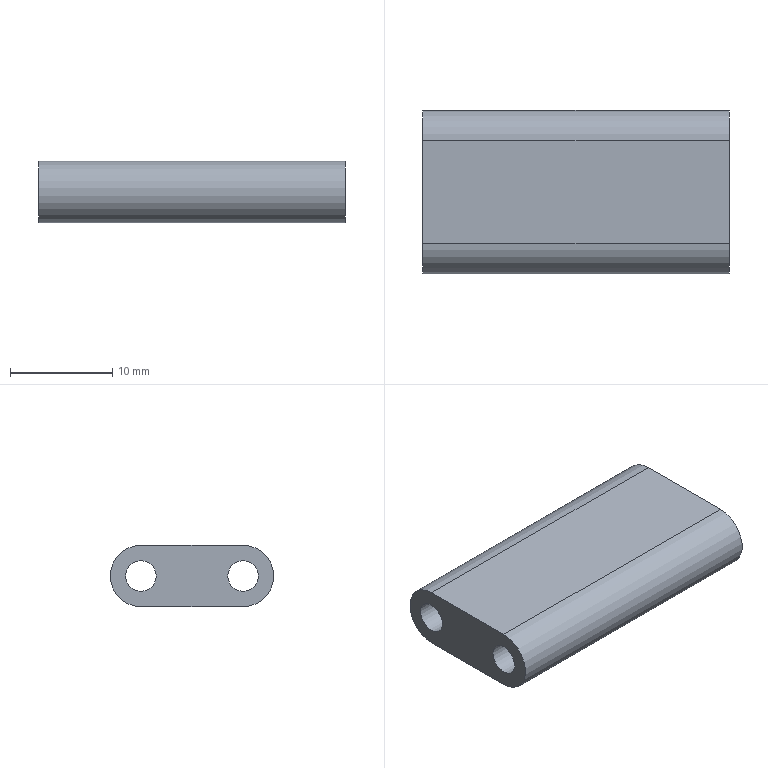Component | NX | PART_4_2 | 1 solid | 8 faces | box 30 x 16 x 6 mm | volume 2224 mm3 | cylinder 4 | plane 4 | commonest cylinder face diameters 6 x2 3 x2
STEP:
#1=CARTESIAN_POINT('',(0.,0.,0.));
#2=DIRECTION('',(0.,0.,1.));
#3=DIRECTION('',(1.,0.,0.));
#4=AXIS2_PLACEMENT_3D('',#1,#2,#3);
#5=CARTESIAN_POINT('',(-15.,1.,103.));
#6=VERTEX_POINT('',#5);
#7=CARTESIAN_POINT('',(-15.,1.,97.));
#8=VERTEX_POINT('',#7);
#9=CARTESIAN_POINT('',(-15.,1.,100.));
#10=DIRECTION('',(1.,0.,0.));
#11=DIRECTION('',(0.,1.,0.));
#12=AXIS2_PLACEMENT_3D('',#9,#10,#11);
#13=CIRCLE('',#12,3.);
#14=CARTESIAN_POINT('',(15.,1.,100.));
#15=DIRECTION('',(-1.,0.,0.));
#16=DIRECTION('',(0.,0.,1.));
#17=AXIS2_PLACEMENT_3D('',#14,#15,#16);
#18=CYLINDRICAL_SURFACE('',#17,3.);
#19=CARTESIAN_POINT('',(7.854,30.));
#20=DIRECTION('',(-1.,0.));
#21=VECTOR('',#20,1.);
#22=LINE('',#19,#21);
#23=(GEOMETRIC_REPRESENTATION_CONTEXT(2)PARAMETRIC_REPRESENTATION_CONTEXT()REPRESENTATION_CONTEXT('',''));
#24=DEFINITIONAL_REPRESENTATION('',(#22),#23);
#25=PCURVE('',#18,#24);
#26=CARTESIAN_POINT('',(-15.,1.,100.));
#27=DIRECTION('',(1.,0.,0.));
#28=DIRECTION('',(0.,0.,-1.));
#29=AXIS2_PLACEMENT_3D('',#26,#27,#28);
#30=PLANE('',#29);
#31=CARTESIAN_POINT('',(0.,0.));
#32=DIRECTION('',(0.,1.));
#33=AXIS2_PLACEMENT_2D('',#31,#32);
#34=CIRCLE('',#33,3.);
#35=(GEOMETRIC_REPRESENTATION_CONTEXT(2)PARAMETRIC_REPRESENTATION_CONTEXT()REPRESENTATION_CONTEXT('',''));
#36=DEFINITIONAL_REPRESENTATION('',(#34),#35);
#37=PCURVE('',#30,#36);
#38=SURFACE_CURVE('',#13,(#25,#37),.PCURVE_S1.);
#39=EDGE_CURVE('',#6,#8,#38,.T.);
#40=ORIENTED_EDGE('',*,*,#39,.T.);
#41=CARTESIAN_POINT('',(15.,1.,97.));
#42=VERTEX_POINT('',#41);
#43=CARTESIAN_POINT('',(15.,1.,97.));
#44=DIRECTION('',(-1.,0.,0.));
#45=VECTOR('',#44,1.);
#46=LINE('',#43,#45);
#47=CARTESIAN_POINT('',(3.142,0.));
#48=DIRECTION('',(0.,1.));
#49=VECTOR('',#48,1.);
#50=LINE('',#47,#49);
#51=(GEOMETRIC_REPRESENTATION_CONTEXT(2)PARAMETRIC_REPRESENTATION_CONTEXT()REPRESENTATION_CONTEXT('',''));
#52=DEFINITIONAL_REPRESENTATION('',(#50),#51);
#53=PCURVE('',#18,#52);
#54=CARTESIAN_POINT('',(15.,1.,97.));
#55=DIRECTION('',(0.,0.,1.));
#56=DIRECTION('',(1.,0.,0.));
#57=AXIS2_PLACEMENT_3D('',#54,#55,#56);
#58=PLANE('',#57);
#59=CARTESIAN_POINT('',(0.,0.));
#60=DIRECTION('',(-1.,0.));
#61=VECTOR('',#60,1.);
#62=LINE('',#59,#61);
#63=(GEOMETRIC_REPRESENTATION_CONTEXT(2)PARAMETRIC_REPRESENTATION_CONTEXT()REPRESENTATION_CONTEXT('',''));
#64=DEFINITIONAL_REPRESENTATION('',(#62),#63);
#65=PCURVE('',#58,#64);
#66=SURFACE_CURVE('',#46,(#53,#65),.PCURVE_S1.);
#67=EDGE_CURVE('',#42,#8,#66,.T.);
#68=ORIENTED_EDGE('',*,*,#67,.F.);
#69=CARTESIAN_POINT('',(15.,1.,103.));
#70=VERTEX_POINT('',#69);
#71=CARTESIAN_POINT('',(15.,1.,100.));
#72=DIRECTION('',(1.,0.,0.));
#73=DIRECTION('',(0.,1.,0.));
#74=AXIS2_PLACEMENT_3D('',#71,#72,#73);
#75=CIRCLE('',#74,3.);
#76=CARTESIAN_POINT('',(7.854,0.));
#77=DIRECTION('',(-1.,0.));
#78=VECTOR('',#77,1.);
#79=LINE('',#76,#78);
#80=(GEOMETRIC_REPRESENTATION_CONTEXT(2)PARAMETRIC_REPRESENTATION_CONTEXT()REPRESENTATION_CONTEXT('',''));
#81=DEFINITIONAL_REPRESENTATION('',(#79),#80);
#82=PCURVE('',#18,#81);
#83=CARTESIAN_POINT('',(15.,1.,100.));
#84=DIRECTION('',(1.,0.,0.));
#85=DIRECTION('',(0.,0.,-1.));
#86=AXIS2_PLACEMENT_3D('',#83,#84,#85);
#87=PLANE('',#86);
#88=CARTESIAN_POINT('',(0.,0.));
#89=DIRECTION('',(0.,1.));
#90=AXIS2_PLACEMENT_2D('',#88,#89);
#91=CIRCLE('',#90,3.);
#92=(GEOMETRIC_REPRESENTATION_CONTEXT(2)PARAMETRIC_REPRESENTATION_CONTEXT()REPRESENTATION_CONTEXT('',''));
#93=DEFINITIONAL_REPRESENTATION('',(#91),#92);
#94=PCURVE('',#87,#93);
#95=SURFACE_CURVE('',#75,(#82,#94),.PCURVE_S1.);
#96=EDGE_CURVE('',#70,#42,#95,.T.);
#97=ORIENTED_EDGE('',*,*,#96,.F.);
#98=CARTESIAN_POINT('',(15.,1.,103.));
#99=DIRECTION('',(-1.,0.,0.));
#100=VECTOR('',#99,1.);
#101=LINE('',#98,#100);
#102=CARTESIAN_POINT('',(6.283,0.));
#103=DIRECTION('',(0.,1.));
#104=VECTOR('',#103,1.);
#105=LINE('',#102,#104);
#106=(GEOMETRIC_REPRESENTATION_CONTEXT(2)PARAMETRIC_REPRESENTATION_CONTEXT()REPRESENTATION_CONTEXT('',''));
#107=DEFINITIONAL_REPRESENTATION('',(#105),#106);
#108=PCURVE('',#18,#107);
#109=CARTESIAN_POINT('',(15.,11.,103.));
#110=DIRECTION('',(0.,0.,-1.));
#111=DIRECTION('',(-1.,0.,0.));
#112=AXIS2_PLACEMENT_3D('',#109,#110,#111);
#113=PLANE('',#112);
#114=CARTESIAN_POINT('',(0.,-10.));
#115=DIRECTION('',(1.,0.));
#116=VECTOR('',#115,1.);
#117=LINE('',#114,#116);
#118=(GEOMETRIC_REPRESENTATION_CONTEXT(2)PARAMETRIC_REPRESENTATION_CONTEXT()REPRESENTATION_CONTEXT('',''));
#119=DEFINITIONAL_REPRESENTATION('',(#117),#118);
#120=PCURVE('',#113,#119);
#121=SURFACE_CURVE('',#101,(#108,#120),.PCURVE_S1.);
#122=EDGE_CURVE('',#70,#6,#121,.T.);
#123=ORIENTED_EDGE('',*,*,#122,.T.);
#124=EDGE_LOOP('',(#40,#68,#97,#123));
#125=FACE_BOUND('',#124,.T.);
#126=ADVANCED_FACE('',(#125),#18,.T.);
#127=CARTESIAN_POINT('',(-15.,11.,97.));
#128=VERTEX_POINT('',#127);
#129=CARTESIAN_POINT('',(-15.,1.,97.));
#130=DIRECTION('',(0.,1.,0.));
#131=VECTOR('',#130,1.);
#132=LINE('',#129,#131);
#133=CARTESIAN_POINT('',(-30.,0.));
#134=DIRECTION('',(0.,1.));
#135=VECTOR('',#134,1.);
#136=LINE('',#133,#135);
#137=(GEOMETRIC_REPRESENTATION_CONTEXT(2)PARAMETRIC_REPRESENTATION_CONTEXT()REPRESENTATION_CONTEXT('',''));
#138=DEFINITIONAL_REPRESENTATION('',(#136),#137);
#139=PCURVE('',#58,#138);
#140=CARTESIAN_POINT('',(3.,0.));
#141=DIRECTION('',(0.,1.));
#142=VECTOR('',#141,1.);
#143=LINE('',#140,#142);
#144=(GEOMETRIC_REPRESENTATION_CONTEXT(2)PARAMETRIC_REPRESENTATION_CONTEXT()REPRESENTATION_CONTEXT('',''));
#145=DEFINITIONAL_REPRESENTATION('',(#143),#144);
#146=PCURVE('',#30,#145);
#147=SURFACE_CURVE('',#132,(#139,#146),.PCURVE_S1.);
#148=EDGE_CURVE('',#8,#128,#147,.T.);
#149=ORIENTED_EDGE('',*,*,#148,.T.);
#150=CARTESIAN_POINT('',(15.,11.,97.));
#151=VERTEX_POINT('',#150);
#152=CARTESIAN_POINT('',(15.,11.,97.));
#153=DIRECTION('',(-1.,0.,0.));
#154=VECTOR('',#153,1.);
#155=LINE('',#152,#154);
#156=CARTESIAN_POINT('',(0.,10.));
#157=DIRECTION('',(-1.,0.));
#158=VECTOR('',#157,1.);
#159=LINE('',#156,#158);
#160=(GEOMETRIC_REPRESENTATION_CONTEXT(2)PARAMETRIC_REPRESENTATION_CONTEXT()REPRESENTATION_CONTEXT('',''));
#161=DEFINITIONAL_REPRESENTATION('',(#159),#160);
#162=PCURVE('',#58,#161);
#163=CARTESIAN_POINT('',(15.,11.,100.));
#164=DIRECTION('',(-1.,0.,0.));
#165=DIRECTION('',(0.,0.,1.));
#166=AXIS2_PLACEMENT_3D('',#163,#164,#165);
#167=CYLINDRICAL_SURFACE('',#166,3.);
#168=CARTESIAN_POINT('',(3.142,0.));
#169=DIRECTION('',(0.,1.));
#170=VECTOR('',#169,1.);
#171=LINE('',#168,#170);
#172=(GEOMETRIC_REPRESENTATION_CONTEXT(2)PARAMETRIC_REPRESENTATION_CONTEXT()REPRESENTATION_CONTEXT('',''));
#173=DEFINITIONAL_REPRESENTATION('',(#171),#172);
#174=PCURVE('',#167,#173);
#175=SURFACE_CURVE('',#155,(#162,#174),.PCURVE_S1.);
#176=EDGE_CURVE('',#151,#128,#175,.T.);
#177=ORIENTED_EDGE('',*,*,#176,.F.);
#178=CARTESIAN_POINT('',(15.,1.,97.));
#179=DIRECTION('',(0.,1.,0.));
#180=VECTOR('',#179,1.);
#181=LINE('',#178,#180);
#182=CARTESIAN_POINT('',(0.,0.));
#183=DIRECTION('',(0.,1.));
#184=VECTOR('',#183,1.);
#185=LINE('',#182,#184);
#186=(GEOMETRIC_REPRESENTATION_CONTEXT(2)PARAMETRIC_REPRESENTATION_CONTEXT()REPRESENTATION_CONTEXT('',''));
#187=DEFINITIONAL_REPRESENTATION('',(#185),#186);
#188=PCURVE('',#58,#187);
#189=CARTESIAN_POINT('',(3.,0.));
#190=DIRECTION('',(0.,1.));
#191=VECTOR('',#190,1.);
#192=LINE('',#189,#191);
#193=(GEOMETRIC_REPRESENTATION_CONTEXT(2)PARAMETRIC_REPRESENTATION_CONTEXT()REPRESENTATION_CONTEXT('',''));
#194=DEFINITIONAL_REPRESENTATION('',(#192),#193);
#195=PCURVE('',#87,#194);
#196=SURFACE_CURVE('',#181,(#188,#195),.PCURVE_S1.);
#197=EDGE_CURVE('',#42,#151,#196,.T.);
#198=ORIENTED_EDGE('',*,*,#197,.F.);
#199=ORIENTED_EDGE('',*,*,#67,.T.);
#200=EDGE_LOOP('',(#149,#177,#198,#199));
#201=FACE_BOUND('',#200,.T.);
#202=ADVANCED_FACE('',(#201),#58,.F.);
#203=CARTESIAN_POINT('',(-15.,11.,103.));
#204=VERTEX_POINT('',#203);
#205=CARTESIAN_POINT('',(-15.,11.,100.));
#206=DIRECTION('',(1.,0.,0.));
#207=DIRECTION('',(0.,1.,0.));
#208=AXIS2_PLACEMENT_3D('',#205,#206,#207);
#209=CIRCLE('',#208,3.);
#210=CARTESIAN_POINT('',(7.854,30.));
#211=DIRECTION('',(-1.,0.));
#212=VECTOR('',#211,1.);
#213=LINE('',#210,#212);
#214=(GEOMETRIC_REPRESENTATION_CONTEXT(2)PARAMETRIC_REPRESENTATION_CONTEXT()REPRESENTATION_CONTEXT('',''));
#215=DEFINITIONAL_REPRESENTATION('',(#213),#214);
#216=PCURVE('',#167,#215);
#217=CARTESIAN_POINT('',(0.,10.));
#218=DIRECTION('',(0.,1.));
#219=AXIS2_PLACEMENT_2D('',#217,#218);
#220=CIRCLE('',#219,3.);
#221=(GEOMETRIC_REPRESENTATION_CONTEXT(2)PARAMETRIC_REPRESENTATION_CONTEXT()REPRESENTATION_CONTEXT('',''));
#222=DEFINITIONAL_REPRESENTATION('',(#220),#221);
#223=PCURVE('',#30,#222);
#224=SURFACE_CURVE('',#209,(#216,#223),.PCURVE_S1.);
#225=EDGE_CURVE('',#128,#204,#224,.T.);
#226=ORIENTED_EDGE('',*,*,#225,.T.);
#227=CARTESIAN_POINT('',(15.,11.,103.));
#228=VERTEX_POINT('',#227);
#229=CARTESIAN_POINT('',(15.,11.,103.));
#230=DIRECTION('',(-1.,0.,0.));
#231=VECTOR('',#230,1.);
#232=LINE('',#229,#231);
#233=CARTESIAN_POINT('',(0.,0.));
#234=DIRECTION('',(0.,1.));
#235=VECTOR('',#234,1.);
#236=LINE('',#233,#235);
#237=(GEOMETRIC_REPRESENTATION_CONTEXT(2)PARAMETRIC_REPRESENTATION_CONTEXT()REPRESENTATION_CONTEXT('',''));
#238=DEFINITIONAL_REPRESENTATION('',(#236),#237);
#239=PCURVE('',#167,#238);
#240=CARTESIAN_POINT('',(0.,0.));
#241=DIRECTION('',(1.,0.));
#242=VECTOR('',#241,1.);
#243=LINE('',#240,#242);
#244=(GEOMETRIC_REPRESENTATION_CONTEXT(2)PARAMETRIC_REPRESENTATION_CONTEXT()REPRESENTATION_CONTEXT('',''));
#245=DEFINITIONAL_REPRESENTATION('',(#243),#244);
#246=PCURVE('',#113,#245);
#247=SURFACE_CURVE('',#232,(#239,#246),.PCURVE_S1.);
#248=EDGE_CURVE('',#228,#204,#247,.T.);
#249=ORIENTED_EDGE('',*,*,#248,.F.);
#250=CARTESIAN_POINT('',(15.,11.,100.));
#251=DIRECTION('',(1.,0.,0.));
#252=DIRECTION('',(0.,1.,0.));
#253=AXIS2_PLACEMENT_3D('',#250,#251,#252);
#254=CIRCLE('',#253,3.);
#255=CARTESIAN_POINT('',(7.854,0.));
#256=DIRECTION('',(-1.,0.));
#257=VECTOR('',#256,1.);
#258=LINE('',#255,#257);
#259=(GEOMETRIC_REPRESENTATION_CONTEXT(2)PARAMETRIC_REPRESENTATION_CONTEXT()REPRESENTATION_CONTEXT('',''));
#260=DEFINITIONAL_REPRESENTATION('',(#258),#259);
#261=PCURVE('',#167,#260);
#262=CARTESIAN_POINT('',(0.,10.));
#263=DIRECTION('',(0.,1.));
#264=AXIS2_PLACEMENT_2D('',#262,#263);
#265=CIRCLE('',#264,3.);
#266=(GEOMETRIC_REPRESENTATION_CONTEXT(2)PARAMETRIC_REPRESENTATION_CONTEXT()REPRESENTATION_CONTEXT('',''));
#267=DEFINITIONAL_REPRESENTATION('',(#265),#266);
#268=PCURVE('',#87,#267);
#269=SURFACE_CURVE('',#254,(#261,#268),.PCURVE_S1.);
#270=EDGE_CURVE('',#151,#228,#269,.T.);
#271=ORIENTED_EDGE('',*,*,#270,.F.);
#272=ORIENTED_EDGE('',*,*,#176,.T.);
#273=EDGE_LOOP('',(#226,#249,#271,#272));
#274=FACE_BOUND('',#273,.T.);
#275=ADVANCED_FACE('',(#274),#167,.T.);
#276=CARTESIAN_POINT('',(15.,2.5,100.));
#277=VERTEX_POINT('',#276);
#278=CARTESIAN_POINT('',(15.,1.,100.));
#279=DIRECTION('',(1.,0.,0.));
#280=DIRECTION('',(0.,1.,0.));
#281=AXIS2_PLACEMENT_3D('',#278,#279,#280);
#282=CIRCLE('',#281,1.5);
#283=CARTESIAN_POINT('',(15.,1.,100.));
#284=DIRECTION('',(-1.,0.,0.));
#285=DIRECTION('',(0.,0.,1.));
#286=AXIS2_PLACEMENT_3D('',#283,#284,#285);
#287=CYLINDRICAL_SURFACE('',#286,1.5);
#288=CARTESIAN_POINT('',(7.854,0.));
#289=DIRECTION('',(-1.,0.));
#290=VECTOR('',#289,1.);
#291=LINE('',#288,#290);
#292=(GEOMETRIC_REPRESENTATION_CONTEXT(2)PARAMETRIC_REPRESENTATION_CONTEXT()REPRESENTATION_CONTEXT('',''));
#293=DEFINITIONAL_REPRESENTATION('',(#291),#292);
#294=PCURVE('',#287,#293);
#295=CARTESIAN_POINT('',(0.,0.));
#296=DIRECTION('',(0.,1.));
#297=AXIS2_PLACEMENT_2D('',#295,#296);
#298=CIRCLE('',#297,1.5);
#299=(GEOMETRIC_REPRESENTATION_CONTEXT(2)PARAMETRIC_REPRESENTATION_CONTEXT()REPRESENTATION_CONTEXT('',''));
#300=DEFINITIONAL_REPRESENTATION('',(#298),#299);
#301=PCURVE('',#87,#300);
#302=SURFACE_CURVE('',#282,(#294,#301),.PCURVE_S1.);
#303=EDGE_CURVE('',#277,#277,#302,.T.);
#304=ORIENTED_EDGE('',*,*,#303,.F.);
#305=CARTESIAN_POINT('',(-15.,2.5,100.));
#306=VERTEX_POINT('',#305);
#307=CARTESIAN_POINT('',(15.,2.5,100.));
#308=CARTESIAN_POINT('',(-15.,2.5,100.));
#309=B_SPLINE_CURVE_WITH_KNOTS('',1,(#307,#308),.UNSPECIFIED.,.F.,.F.,(2,2),(0.,30.),.PIECEWISE_BEZIER_KNOTS.);
#310=CARTESIAN_POINT('',(7.854,0.));
#311=DIRECTION('',(0.,1.));
#312=VECTOR('',#311,1.);
#313=LINE('',#310,#312);
#314=(GEOMETRIC_REPRESENTATION_CONTEXT(2)PARAMETRIC_REPRESENTATION_CONTEXT()REPRESENTATION_CONTEXT('',''));
#315=DEFINITIONAL_REPRESENTATION('',(#313),#314);
#316=PCURVE('',#287,#315);
#317=CARTESIAN_POINT('',(1.571,0.));
#318=DIRECTION('',(0.,1.));
#319=VECTOR('',#318,1.);
#320=LINE('',#317,#319);
#321=(GEOMETRIC_REPRESENTATION_CONTEXT(2)PARAMETRIC_REPRESENTATION_CONTEXT()REPRESENTATION_CONTEXT('',''));
#322=DEFINITIONAL_REPRESENTATION('',(#320),#321);
#323=PCURVE('',#287,#322);
#324=SEAM_CURVE('',#309,(#316,#323),.PCURVE_S1.);
#325=EDGE_CURVE('',#277,#306,#324,.T.);
#326=ORIENTED_EDGE('',*,*,#325,.T.);
#327=CARTESIAN_POINT('',(-15.,1.,100.));
#328=DIRECTION('',(1.,0.,0.));
#329=DIRECTION('',(0.,1.,0.));
#330=AXIS2_PLACEMENT_3D('',#327,#328,#329);
#331=CIRCLE('',#330,1.5);
#332=CARTESIAN_POINT('',(7.854,30.));
#333=DIRECTION('',(-1.,0.));
#334=VECTOR('',#333,1.);
#335=LINE('',#332,#334);
#336=(GEOMETRIC_REPRESENTATION_CONTEXT(2)PARAMETRIC_REPRESENTATION_CONTEXT()REPRESENTATION_CONTEXT('',''));
#337=DEFINITIONAL_REPRESENTATION('',(#335),#336);
#338=PCURVE('',#287,#337);
#339=CARTESIAN_POINT('',(0.,0.));
#340=DIRECTION('',(0.,1.));
#341=AXIS2_PLACEMENT_2D('',#339,#340);
#342=CIRCLE('',#341,1.5);
#343=(GEOMETRIC_REPRESENTATION_CONTEXT(2)PARAMETRIC_REPRESENTATION_CONTEXT()REPRESENTATION_CONTEXT('',''));
#344=DEFINITIONAL_REPRESENTATION('',(#342),#343);
#345=PCURVE('',#30,#344);
#346=SURFACE_CURVE('',#331,(#338,#345),.PCURVE_S1.);
#347=EDGE_CURVE('',#306,#306,#346,.T.);
#348=ORIENTED_EDGE('',*,*,#347,.T.);
#349=ORIENTED_EDGE('',*,*,#325,.F.);
#350=EDGE_LOOP('',(#304,#326,#348,#349));
#351=FACE_BOUND('',#350,.F.);
#352=ADVANCED_FACE('',(#351),#287,.F.);
#353=CARTESIAN_POINT('',(-15.,11.,103.));
#354=DIRECTION('',(0.,-1.,0.));
#355=VECTOR('',#354,1.);
#356=LINE('',#353,#355);
#357=CARTESIAN_POINT('',(30.,0.));
#358=DIRECTION('',(0.,-1.));
#359=VECTOR('',#358,1.);
#360=LINE('',#357,#359);
#361=(GEOMETRIC_REPRESENTATION_CONTEXT(2)PARAMETRIC_REPRESENTATION_CONTEXT()REPRESENTATION_CONTEXT('',''));
#362=DEFINITIONAL_REPRESENTATION('',(#360),#361);
#363=PCURVE('',#113,#362);
#364=CARTESIAN_POINT('',(-3.,10.));
#365=DIRECTION('',(0.,-1.));
#366=VECTOR('',#365,1.);
#367=LINE('',#364,#366);
#368=(GEOMETRIC_REPRESENTATION_CONTEXT(2)PARAMETRIC_REPRESENTATION_CONTEXT()REPRESENTATION_CONTEXT('',''));
#369=DEFINITIONAL_REPRESENTATION('',(#367),#368);
#370=PCURVE('',#30,#369);
#371=SURFACE_CURVE('',#356,(#363,#370),.PCURVE_S1.);
#372=EDGE_CURVE('',#204,#6,#371,.T.);
#373=ORIENTED_EDGE('',*,*,#372,.T.);
#374=ORIENTED_EDGE('',*,*,#122,.F.);
#375=CARTESIAN_POINT('',(15.,11.,103.));
#376=DIRECTION('',(0.,-1.,0.));
#377=VECTOR('',#376,1.);
#378=LINE('',#375,#377);
#379=CARTESIAN_POINT('',(0.,0.));
#380=DIRECTION('',(0.,-1.));
#381=VECTOR('',#380,1.);
#382=LINE('',#379,#381);
#383=(GEOMETRIC_REPRESENTATION_CONTEXT(2)PARAMETRIC_REPRESENTATION_CONTEXT()REPRESENTATION_CONTEXT('',''));
#384=DEFINITIONAL_REPRESENTATION('',(#382),#383);
#385=PCURVE('',#113,#384);
#386=CARTESIAN_POINT('',(-3.,10.));
#387=DIRECTION('',(0.,-1.));
#388=VECTOR('',#387,1.);
#389=LINE('',#386,#388);
#390=(GEOMETRIC_REPRESENTATION_CONTEXT(2)PARAMETRIC_REPRESENTATION_CONTEXT()REPRESENTATION_CONTEXT('',''));
#391=DEFINITIONAL_REPRESENTATION('',(#389),#390);
#392=PCURVE('',#87,#391);
#393=SURFACE_CURVE('',#378,(#385,#392),.PCURVE_S1.);
#394=EDGE_CURVE('',#228,#70,#393,.T.);
#395=ORIENTED_EDGE('',*,*,#394,.F.);
#396=ORIENTED_EDGE('',*,*,#248,.T.);
#397=EDGE_LOOP('',(#373,#374,#395,#396));
#398=FACE_BOUND('',#397,.T.);
#399=ADVANCED_FACE('',(#398),#113,.F.);
#400=CARTESIAN_POINT('',(15.,12.5,100.));
#401=VERTEX_POINT('',#400);
#402=CARTESIAN_POINT('',(15.,11.,100.));
#403=DIRECTION('',(1.,0.,0.));
#404=DIRECTION('',(0.,1.,0.));
#405=AXIS2_PLACEMENT_3D('',#402,#403,#404);
#406=CIRCLE('',#405,1.5);
#407=CARTESIAN_POINT('',(15.,11.,100.));
#408=DIRECTION('',(-1.,0.,0.));
#409=DIRECTION('',(0.,0.,1.));
#410=AXIS2_PLACEMENT_3D('',#407,#408,#409);
#411=CYLINDRICAL_SURFACE('',#410,1.5);
#412=CARTESIAN_POINT('',(7.854,0.));
#413=DIRECTION('',(-1.,0.));
#414=VECTOR('',#413,1.);
#415=LINE('',#412,#414);
#416=(GEOMETRIC_REPRESENTATION_CONTEXT(2)PARAMETRIC_REPRESENTATION_CONTEXT()REPRESENTATION_CONTEXT('',''));
#417=DEFINITIONAL_REPRESENTATION('',(#415),#416);
#418=PCURVE('',#411,#417);
#419=CARTESIAN_POINT('',(0.,10.));
#420=DIRECTION('',(0.,1.));
#421=AXIS2_PLACEMENT_2D('',#419,#420);
#422=CIRCLE('',#421,1.5);
#423=(GEOMETRIC_REPRESENTATION_CONTEXT(2)PARAMETRIC_REPRESENTATION_CONTEXT()REPRESENTATION_CONTEXT('',''));
#424=DEFINITIONAL_REPRESENTATION('',(#422),#423);
#425=PCURVE('',#87,#424);
#426=SURFACE_CURVE('',#406,(#418,#425),.PCURVE_S1.);
#427=EDGE_CURVE('',#401,#401,#426,.T.);
#428=ORIENTED_EDGE('',*,*,#427,.F.);
#429=CARTESIAN_POINT('',(-15.,12.5,100.));
#430=VERTEX_POINT('',#429);
#431=CARTESIAN_POINT('',(15.,12.5,100.));
#432=CARTESIAN_POINT('',(-15.,12.5,100.));
#433=B_SPLINE_CURVE_WITH_KNOTS('',1,(#431,#432),.UNSPECIFIED.,.F.,.F.,(2,2),(0.,30.),.PIECEWISE_BEZIER_KNOTS.);
#434=CARTESIAN_POINT('',(7.854,0.));
#435=DIRECTION('',(0.,1.));
#436=VECTOR('',#435,1.);
#437=LINE('',#434,#436);
#438=(GEOMETRIC_REPRESENTATION_CONTEXT(2)PARAMETRIC_REPRESENTATION_CONTEXT()REPRESENTATION_CONTEXT('',''));
#439=DEFINITIONAL_REPRESENTATION('',(#437),#438);
#440=PCURVE('',#411,#439);
#441=CARTESIAN_POINT('',(1.571,0.));
#442=DIRECTION('',(0.,1.));
#443=VECTOR('',#442,1.);
#444=LINE('',#441,#443);
#445=(GEOMETRIC_REPRESENTATION_CONTEXT(2)PARAMETRIC_REPRESENTATION_CONTEXT()REPRESENTATION_CONTEXT('',''));
#446=DEFINITIONAL_REPRESENTATION('',(#444),#445);
#447=PCURVE('',#411,#446);
#448=SEAM_CURVE('',#433,(#440,#447),.PCURVE_S1.);
#449=EDGE_CURVE('',#401,#430,#448,.T.);
#450=ORIENTED_EDGE('',*,*,#449,.T.);
#451=CARTESIAN_POINT('',(-15.,11.,100.));
#452=DIRECTION('',(1.,0.,0.));
#453=DIRECTION('',(0.,1.,0.));
#454=AXIS2_PLACEMENT_3D('',#451,#452,#453);
#455=CIRCLE('',#454,1.5);
#456=CARTESIAN_POINT('',(7.854,30.));
#457=DIRECTION('',(-1.,0.));
#458=VECTOR('',#457,1.);
#459=LINE('',#456,#458);
#460=(GEOMETRIC_REPRESENTATION_CONTEXT(2)PARAMETRIC_REPRESENTATION_CONTEXT()REPRESENTATION_CONTEXT('',''));
#461=DEFINITIONAL_REPRESENTATION('',(#459),#460);
#462=PCURVE('',#411,#461);
#463=CARTESIAN_POINT('',(0.,10.));
#464=DIRECTION('',(0.,1.));
#465=AXIS2_PLACEMENT_2D('',#463,#464);
#466=CIRCLE('',#465,1.5);
#467=(GEOMETRIC_REPRESENTATION_CONTEXT(2)PARAMETRIC_REPRESENTATION_CONTEXT()REPRESENTATION_CONTEXT('',''));
#468=DEFINITIONAL_REPRESENTATION('',(#466),#467);
#469=PCURVE('',#30,#468);
#470=SURFACE_CURVE('',#455,(#462,#469),.PCURVE_S1.);
#471=EDGE_CURVE('',#430,#430,#470,.T.);
#472=ORIENTED_EDGE('',*,*,#471,.T.);
#473=ORIENTED_EDGE('',*,*,#449,.F.);
#474=EDGE_LOOP('',(#428,#450,#472,#473));
#475=FACE_BOUND('',#474,.F.);
#476=ADVANCED_FACE('',(#475),#411,.F.);
#477=ORIENTED_EDGE('',*,*,#96,.T.);
#478=ORIENTED_EDGE('',*,*,#197,.T.);
#479=ORIENTED_EDGE('',*,*,#270,.T.);
#480=ORIENTED_EDGE('',*,*,#394,.T.);
#481=EDGE_LOOP('',(#477,#478,#479,#480));
#482=FACE_BOUND('',#481,.T.);
#483=ORIENTED_EDGE('',*,*,#303,.F.);
#484=EDGE_LOOP('',(#483));
#485=FACE_BOUND('',#484,.T.);
#486=ORIENTED_EDGE('',*,*,#427,.F.);
#487=EDGE_LOOP('',(#486));
#488=FACE_BOUND('',#487,.T.);
#489=ADVANCED_FACE('',(#482,#485,#488),#87,.T.);
#490=ORIENTED_EDGE('',*,*,#39,.F.);
#491=ORIENTED_EDGE('',*,*,#372,.F.);
#492=ORIENTED_EDGE('',*,*,#225,.F.);
#493=ORIENTED_EDGE('',*,*,#148,.F.);
#494=EDGE_LOOP('',(#490,#491,#492,#493));
#495=FACE_BOUND('',#494,.T.);
#496=ORIENTED_EDGE('',*,*,#347,.T.);
#497=EDGE_LOOP('',(#496));
#498=FACE_BOUND('',#497,.T.);
#499=ORIENTED_EDGE('',*,*,#471,.T.);
#500=EDGE_LOOP('',(#499));
#501=FACE_BOUND('',#500,.T.);
#502=ADVANCED_FACE('',(#495,#498,#501),#30,.F.);
#503=CLOSED_SHELL('',(#126,#202,#275,#352,#399,#476,#489,#502));
#504=MANIFOLD_SOLID_BREP('',#503);
#505=(LENGTH_UNIT()NAMED_UNIT(*)SI_UNIT(.MILLI.,.METRE.));
#506=UNCERTAINTY_MEASURE_WITH_UNIT(LENGTH_MEASURE(0.000002),#505,'','');
#507=(NAMED_UNIT(*)PLANE_ANGLE_UNIT()SI_UNIT($,.RADIAN.));
#508=(NAMED_UNIT(*)SI_UNIT($,.STERADIAN.)SOLID_ANGLE_UNIT());
#509=(GEOMETRIC_REPRESENTATION_CONTEXT(3)GLOBAL_UNCERTAINTY_ASSIGNED_CONTEXT((#506))GLOBAL_UNIT_ASSIGNED_CONTEXT((#505,#507,#508))REPRESENTATION_CONTEXT('',''));
#510=ADVANCED_BREP_SHAPE_REPRESENTATION('',(#4,#504),#509);